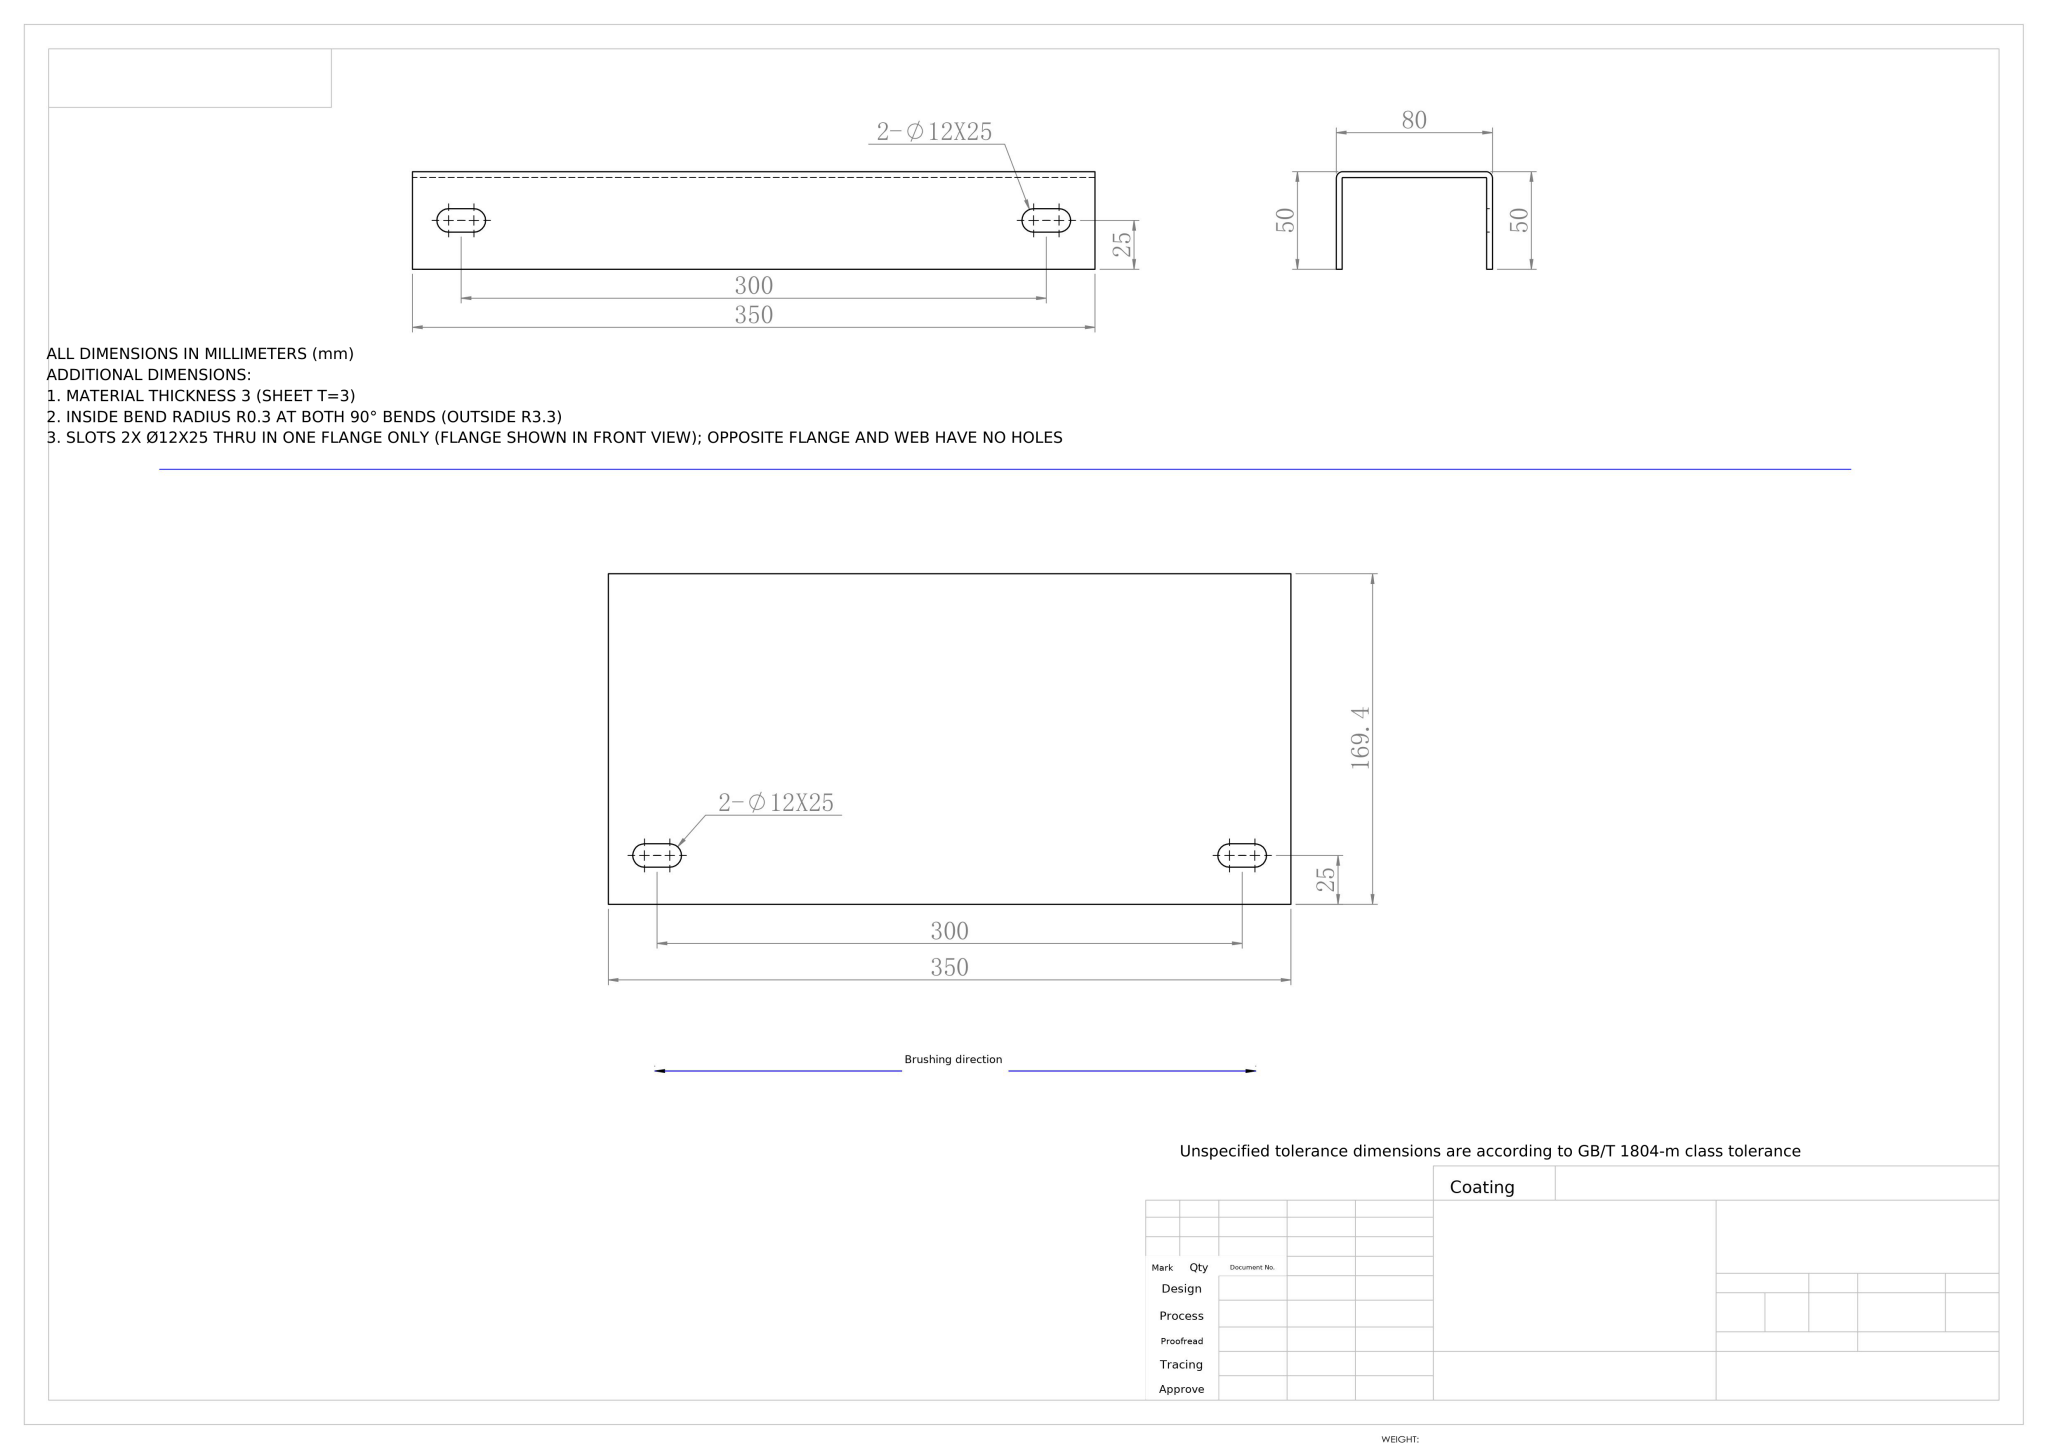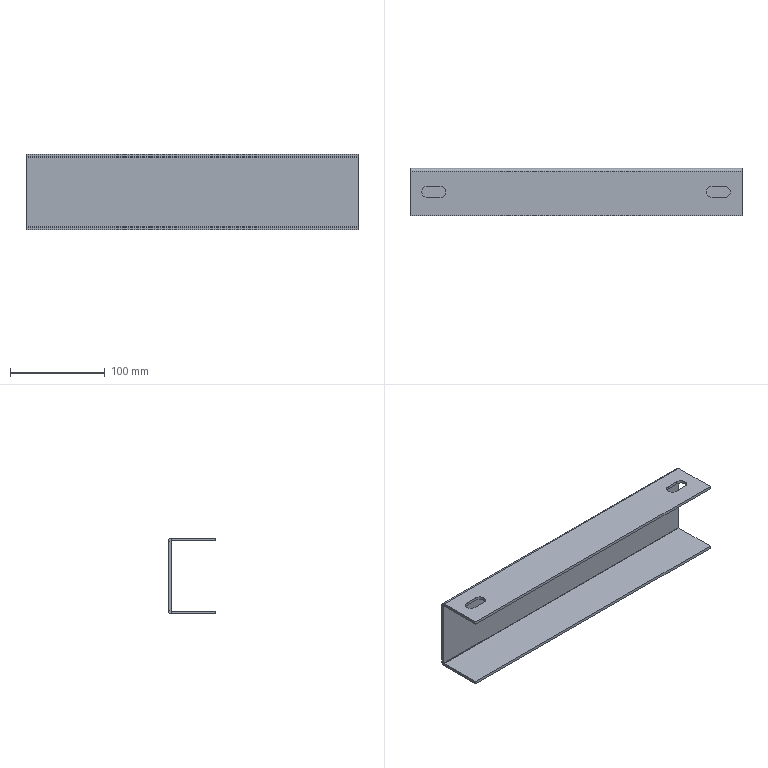Part | NX | mm | 1 solid | 32 faces | box 350 x 50 x 80 mm | volume 179463 mm3 | plane 22 | cylinder 10 | commonest cylinder face diameters 12 x6 6.6 x2 0.6 x2
STEP:
#1=COLOUR_RGB('',0.7529,0.7529,0.7529);
#2=FILL_AREA_STYLE_COLOUR('',#1);
#3=FILL_AREA_STYLE('',(#2));
#4=SURFACE_STYLE_FILL_AREA(#3);
#5=SURFACE_SIDE_STYLE('',(#4));
#6=SURFACE_STYLE_USAGE(.BOTH.,#5);
#7=PRESENTATION_STYLE_ASSIGNMENT((#6));
#8=CARTESIAN_POINT('',(337.5,25.,-3.));
#9=VERTEX_POINT('',#8);
#10=CARTESIAN_POINT('',(331.5,31.,-3.));
#11=VERTEX_POINT('',#10);
#12=CARTESIAN_POINT('',(331.5,25.,-3.));
#13=DIRECTION('',(0.,0.,1.));
#14=DIRECTION('',(-1.,0.,0.));
#15=AXIS2_PLACEMENT_3D('',#12,#13,#14);
#16=CIRCLE('',#15,6.);
#17=EDGE_CURVE('',#9,#11,#16,.T.);
#18=ORIENTED_EDGE('',*,*,#17,.F.);
#19=CARTESIAN_POINT('',(337.5,25.,0.));
#20=VERTEX_POINT('',#19);
#21=CARTESIAN_POINT('',(337.5,25.,-3.));
#22=DIRECTION('',(0.,0.,1.));
#23=VECTOR('',#22,1000.);
#24=LINE('',#21,#23);
#25=EDGE_CURVE('',#9,#20,#24,.T.);
#26=ORIENTED_EDGE('',*,*,#25,.T.);
#27=CARTESIAN_POINT('',(331.5,31.,0.));
#28=VERTEX_POINT('',#27);
#29=CARTESIAN_POINT('',(331.5,25.,0.));
#30=DIRECTION('',(0.,0.,1.));
#31=DIRECTION('',(-1.,0.,0.));
#32=AXIS2_PLACEMENT_3D('',#29,#30,#31);
#33=CIRCLE('',#32,6.);
#34=EDGE_CURVE('',#20,#28,#33,.T.);
#35=ORIENTED_EDGE('',*,*,#34,.T.);
#36=CARTESIAN_POINT('',(331.5,31.,-3.));
#37=DIRECTION('',(0.,0.,1.));
#38=VECTOR('',#37,1000.);
#39=LINE('',#36,#38);
#40=EDGE_CURVE('',#11,#28,#39,.T.);
#41=ORIENTED_EDGE('',*,*,#40,.F.);
#42=EDGE_LOOP('',(#18,#26,#35,#41));
#43=FACE_OUTER_BOUND('',#42,.T.);
#44=CARTESIAN_POINT('',(331.5,25.,-3.));
#45=DIRECTION('',(0.,0.,1.));
#46=DIRECTION('',(1.,0.,0.));
#47=AXIS2_PLACEMENT_3D('',#44,#45,#46);
#48=CYLINDRICAL_SURFACE('',#47,6.);
#49=ADVANCED_FACE('',(#43),#48,.F.);
#50=CARTESIAN_POINT('',(37.5,25.,-3.));
#51=VERTEX_POINT('',#50);
#52=CARTESIAN_POINT('',(31.5,31.,-3.));
#53=VERTEX_POINT('',#52);
#54=CARTESIAN_POINT('',(31.5,25.,-3.));
#55=DIRECTION('',(0.,0.,1.));
#56=DIRECTION('',(-1.,0.,0.));
#57=AXIS2_PLACEMENT_3D('',#54,#55,#56);
#58=CIRCLE('',#57,6.);
#59=EDGE_CURVE('',#51,#53,#58,.T.);
#60=ORIENTED_EDGE('',*,*,#59,.F.);
#61=CARTESIAN_POINT('',(37.5,25.,0.));
#62=VERTEX_POINT('',#61);
#63=CARTESIAN_POINT('',(37.5,25.,-3.));
#64=DIRECTION('',(0.,0.,1.));
#65=VECTOR('',#64,1000.);
#66=LINE('',#63,#65);
#67=EDGE_CURVE('',#51,#62,#66,.T.);
#68=ORIENTED_EDGE('',*,*,#67,.T.);
#69=CARTESIAN_POINT('',(31.5,31.,0.));
#70=VERTEX_POINT('',#69);
#71=CARTESIAN_POINT('',(31.5,25.,0.));
#72=DIRECTION('',(0.,0.,1.));
#73=DIRECTION('',(-1.,0.,0.));
#74=AXIS2_PLACEMENT_3D('',#71,#72,#73);
#75=CIRCLE('',#74,6.);
#76=EDGE_CURVE('',#62,#70,#75,.T.);
#77=ORIENTED_EDGE('',*,*,#76,.T.);
#78=CARTESIAN_POINT('',(31.5,31.,-3.));
#79=DIRECTION('',(0.,0.,1.));
#80=VECTOR('',#79,1000.);
#81=LINE('',#78,#80);
#82=EDGE_CURVE('',#53,#70,#81,.T.);
#83=ORIENTED_EDGE('',*,*,#82,.F.);
#84=EDGE_LOOP('',(#60,#68,#77,#83));
#85=FACE_OUTER_BOUND('',#84,.T.);
#86=CARTESIAN_POINT('',(31.5,25.,-3.));
#87=DIRECTION('',(0.,0.,1.));
#88=DIRECTION('',(1.,0.,0.));
#89=AXIS2_PLACEMENT_3D('',#86,#87,#88);
#90=CYLINDRICAL_SURFACE('',#89,6.);
#91=ADVANCED_FACE('',(#85),#90,.F.);
#92=CARTESIAN_POINT('',(350.,50.,-3.3));
#93=VERTEX_POINT('',#92);
#94=CARTESIAN_POINT('',(350.,47.,-3.3));
#95=VERTEX_POINT('',#94);
#96=CARTESIAN_POINT('',(350.,50.,-3.3));
#97=DIRECTION('',(0.,-1.,0.));
#98=VECTOR('',#97,1000.);
#99=LINE('',#96,#98);
#100=EDGE_CURVE('',#93,#95,#99,.T.);
#101=ORIENTED_EDGE('',*,*,#100,.F.);
#102=CARTESIAN_POINT('',(350.,46.7,0.));
#103=VERTEX_POINT('',#102);
#104=CARTESIAN_POINT('',(350.,46.7,-3.3));
#105=DIRECTION('',(-1.,0.,0.));
#106=DIRECTION('',(0.,0.,-1.));
#107=AXIS2_PLACEMENT_3D('',#104,#105,#106);
#108=CIRCLE('',#107,3.3);
#109=EDGE_CURVE('',#103,#93,#108,.T.);
#110=ORIENTED_EDGE('',*,*,#109,.F.);
#111=CARTESIAN_POINT('',(350.,46.7,-3.));
#112=VERTEX_POINT('',#111);
#113=CARTESIAN_POINT('',(350.,46.7,-3.));
#114=DIRECTION('',(0.,0.,1.));
#115=VECTOR('',#114,1000.);
#116=LINE('',#113,#115);
#117=EDGE_CURVE('',#112,#103,#116,.T.);
#118=ORIENTED_EDGE('',*,*,#117,.F.);
#119=CARTESIAN_POINT('',(350.,46.7,-3.3));
#120=DIRECTION('',(-1.,0.,0.));
#121=DIRECTION('',(0.,0.,-1.));
#122=AXIS2_PLACEMENT_3D('',#119,#120,#121);
#123=CIRCLE('',#122,0.3);
#124=EDGE_CURVE('',#112,#95,#123,.T.);
#125=ORIENTED_EDGE('',*,*,#124,.T.);
#126=EDGE_LOOP('',(#101,#110,#118,#125));
#127=FACE_OUTER_BOUND('',#126,.T.);
#128=CARTESIAN_POINT('',(350.,50.,-3.3));
#129=DIRECTION('',(1.,0.,0.));
#130=DIRECTION('',(0.,0.,-1.));
#131=AXIS2_PLACEMENT_3D('',#128,#129,#130);
#132=PLANE('',#131);
#133=ADVANCED_FACE('',(#127),#132,.T.);
#134=CARTESIAN_POINT('',(350.,50.,-76.7));
#135=VERTEX_POINT('',#134);
#136=CARTESIAN_POINT('',(350.,50.,0.));
#137=DIRECTION('',(0.,0.,-1.));
#138=VECTOR('',#137,1000.);
#139=LINE('',#136,#138);
#140=EDGE_CURVE('',#93,#135,#139,.T.);
#141=ORIENTED_EDGE('',*,*,#140,.F.);
#142=ORIENTED_EDGE('',*,*,#100,.T.);
#143=CARTESIAN_POINT('',(350.,47.,-76.7));
#144=VERTEX_POINT('',#143);
#145=CARTESIAN_POINT('',(350.,47.,0.));
#146=DIRECTION('',(0.,0.,-1.));
#147=VECTOR('',#146,1000.);
#148=LINE('',#145,#147);
#149=EDGE_CURVE('',#95,#144,#148,.T.);
#150=ORIENTED_EDGE('',*,*,#149,.T.);
#151=CARTESIAN_POINT('',(350.,47.,-76.7));
#152=DIRECTION('',(0.,1.,0.));
#153=VECTOR('',#152,1000.);
#154=LINE('',#151,#153);
#155=EDGE_CURVE('',#144,#135,#154,.T.);
#156=ORIENTED_EDGE('',*,*,#155,.T.);
#157=EDGE_LOOP('',(#141,#142,#150,#156));
#158=FACE_OUTER_BOUND('',#157,.T.);
#159=CARTESIAN_POINT('',(350.,46.7,-3.));
#160=DIRECTION('',(1.,0.,0.));
#161=DIRECTION('',(0.,0.,-1.));
#162=AXIS2_PLACEMENT_3D('',#159,#160,#161);
#163=PLANE('',#162);
#164=ADVANCED_FACE('',(#158),#163,.T.);
#165=CARTESIAN_POINT('',(0.,46.7,0.));
#166=VERTEX_POINT('',#165);
#167=CARTESIAN_POINT('',(0.,46.7,-3.));
#168=VERTEX_POINT('',#167);
#169=CARTESIAN_POINT('',(0.,46.7,0.));
#170=DIRECTION('',(0.,0.,-1.));
#171=VECTOR('',#170,1000.);
#172=LINE('',#169,#171);
#173=EDGE_CURVE('',#166,#168,#172,.T.);
#174=ORIENTED_EDGE('',*,*,#173,.F.);
#175=CARTESIAN_POINT('',(0.,50.,-3.3));
#176=VERTEX_POINT('',#175);
#177=CARTESIAN_POINT('',(0.,46.7,-3.3));
#178=DIRECTION('',(-1.,0.,0.));
#179=DIRECTION('',(0.,0.,-1.));
#180=AXIS2_PLACEMENT_3D('',#177,#178,#179);
#181=CIRCLE('',#180,3.3);
#182=EDGE_CURVE('',#166,#176,#181,.T.);
#183=ORIENTED_EDGE('',*,*,#182,.T.);
#184=CARTESIAN_POINT('',(0.,47.,-3.3));
#185=VERTEX_POINT('',#184);
#186=CARTESIAN_POINT('',(0.,47.,-3.3));
#187=DIRECTION('',(0.,1.,0.));
#188=VECTOR('',#187,1000.);
#189=LINE('',#186,#188);
#190=EDGE_CURVE('',#185,#176,#189,.T.);
#191=ORIENTED_EDGE('',*,*,#190,.F.);
#192=CARTESIAN_POINT('',(0.,46.7,-3.3));
#193=DIRECTION('',(-1.,0.,0.));
#194=DIRECTION('',(0.,0.,-1.));
#195=AXIS2_PLACEMENT_3D('',#192,#193,#194);
#196=CIRCLE('',#195,0.3);
#197=EDGE_CURVE('',#168,#185,#196,.T.);
#198=ORIENTED_EDGE('',*,*,#197,.F.);
#199=EDGE_LOOP('',(#174,#183,#191,#198));
#200=FACE_OUTER_BOUND('',#199,.T.);
#201=CARTESIAN_POINT('',(0.,46.7,0.));
#202=DIRECTION('',(-1.,0.,0.));
#203=DIRECTION('',(0.,0.,1.));
#204=AXIS2_PLACEMENT_3D('',#201,#202,#203);
#205=PLANE('',#204);
#206=ADVANCED_FACE('',(#200),#205,.T.);
#207=CARTESIAN_POINT('',(0.,0.,0.));
#208=VERTEX_POINT('',#207);
#209=CARTESIAN_POINT('',(0.,0.,0.));
#210=DIRECTION('',(0.,1.,0.));
#211=VECTOR('',#210,1000.);
#212=LINE('',#209,#211);
#213=EDGE_CURVE('',#208,#166,#212,.T.);
#214=ORIENTED_EDGE('',*,*,#213,.T.);
#215=ORIENTED_EDGE('',*,*,#173,.T.);
#216=CARTESIAN_POINT('',(0.,0.,-3.));
#217=VERTEX_POINT('',#216);
#218=CARTESIAN_POINT('',(0.,0.,-3.));
#219=DIRECTION('',(0.,1.,0.));
#220=VECTOR('',#219,1000.);
#221=LINE('',#218,#220);
#222=EDGE_CURVE('',#217,#168,#221,.T.);
#223=ORIENTED_EDGE('',*,*,#222,.F.);
#224=CARTESIAN_POINT('',(0.,0.,-3.));
#225=DIRECTION('',(0.,0.,1.));
#226=VECTOR('',#225,1000.);
#227=LINE('',#224,#226);
#228=EDGE_CURVE('',#217,#208,#227,.T.);
#229=ORIENTED_EDGE('',*,*,#228,.T.);
#230=EDGE_LOOP('',(#214,#215,#223,#229));
#231=FACE_OUTER_BOUND('',#230,.T.);
#232=CARTESIAN_POINT('',(0.,47.,-3.3));
#233=DIRECTION('',(-1.,0.,0.));
#234=DIRECTION('',(0.,0.,1.));
#235=AXIS2_PLACEMENT_3D('',#232,#233,#234);
#236=PLANE('',#235);
#237=ADVANCED_FACE('',(#231),#236,.T.);
#238=CARTESIAN_POINT('',(350.,46.7,-80.));
#239=VERTEX_POINT('',#238);
#240=CARTESIAN_POINT('',(350.,46.7,-77.));
#241=VERTEX_POINT('',#240);
#242=CARTESIAN_POINT('',(350.,46.7,-80.));
#243=DIRECTION('',(0.,0.,1.));
#244=VECTOR('',#243,1000.);
#245=LINE('',#242,#244);
#246=EDGE_CURVE('',#239,#241,#245,.T.);
#247=ORIENTED_EDGE('',*,*,#246,.F.);
#248=CARTESIAN_POINT('',(350.,46.7,-76.7));
#249=DIRECTION('',(-1.,0.,0.));
#250=DIRECTION('',(0.,0.,-1.));
#251=AXIS2_PLACEMENT_3D('',#248,#249,#250);
#252=CIRCLE('',#251,3.3);
#253=EDGE_CURVE('',#135,#239,#252,.T.);
#254=ORIENTED_EDGE('',*,*,#253,.F.);
#255=ORIENTED_EDGE('',*,*,#155,.F.);
#256=CARTESIAN_POINT('',(350.,46.7,-76.7));
#257=DIRECTION('',(-1.,0.,0.));
#258=DIRECTION('',(0.,0.,-1.));
#259=AXIS2_PLACEMENT_3D('',#256,#257,#258);
#260=CIRCLE('',#259,0.3);
#261=EDGE_CURVE('',#144,#241,#260,.T.);
#262=ORIENTED_EDGE('',*,*,#261,.T.);
#263=EDGE_LOOP('',(#247,#254,#255,#262));
#264=FACE_OUTER_BOUND('',#263,.T.);
#265=CARTESIAN_POINT('',(350.,46.7,-80.));
#266=DIRECTION('',(1.,0.,0.));
#267=DIRECTION('',(0.,0.,-1.));
#268=AXIS2_PLACEMENT_3D('',#265,#266,#267);
#269=PLANE('',#268);
#270=ADVANCED_FACE('',(#264),#269,.T.);
#271=CARTESIAN_POINT('',(350.,0.,-80.));
#272=VERTEX_POINT('',#271);
#273=CARTESIAN_POINT('',(350.,50.,-80.));
#274=DIRECTION('',(0.,-1.,0.));
#275=VECTOR('',#274,1000.);
#276=LINE('',#273,#275);
#277=EDGE_CURVE('',#239,#272,#276,.T.);
#278=ORIENTED_EDGE('',*,*,#277,.F.);
#279=ORIENTED_EDGE('',*,*,#246,.T.);
#280=CARTESIAN_POINT('',(350.,0.,-77.));
#281=VERTEX_POINT('',#280);
#282=CARTESIAN_POINT('',(350.,50.,-77.));
#283=DIRECTION('',(0.,-1.,0.));
#284=VECTOR('',#283,1000.);
#285=LINE('',#282,#284);
#286=EDGE_CURVE('',#241,#281,#285,.T.);
#287=ORIENTED_EDGE('',*,*,#286,.T.);
#288=CARTESIAN_POINT('',(350.,0.,-80.));
#289=DIRECTION('',(0.,0.,1.));
#290=VECTOR('',#289,1000.);
#291=LINE('',#288,#290);
#292=EDGE_CURVE('',#272,#281,#291,.T.);
#293=ORIENTED_EDGE('',*,*,#292,.F.);
#294=EDGE_LOOP('',(#278,#279,#287,#293));
#295=FACE_OUTER_BOUND('',#294,.T.);
#296=CARTESIAN_POINT('',(350.,47.,-76.7));
#297=DIRECTION('',(1.,0.,0.));
#298=DIRECTION('',(0.,0.,-1.));
#299=AXIS2_PLACEMENT_3D('',#296,#297,#298);
#300=PLANE('',#299);
#301=ADVANCED_FACE('',(#295),#300,.T.);
#302=CARTESIAN_POINT('',(0.,50.,-76.7));
#303=VERTEX_POINT('',#302);
#304=CARTESIAN_POINT('',(0.,47.,-76.7));
#305=VERTEX_POINT('',#304);
#306=CARTESIAN_POINT('',(0.,50.,-76.7));
#307=DIRECTION('',(0.,-1.,0.));
#308=VECTOR('',#307,1000.);
#309=LINE('',#306,#308);
#310=EDGE_CURVE('',#303,#305,#309,.T.);
#311=ORIENTED_EDGE('',*,*,#310,.F.);
#312=CARTESIAN_POINT('',(0.,46.7,-80.));
#313=VERTEX_POINT('',#312);
#314=CARTESIAN_POINT('',(0.,46.7,-76.7));
#315=DIRECTION('',(-1.,0.,0.));
#316=DIRECTION('',(0.,0.,-1.));
#317=AXIS2_PLACEMENT_3D('',#314,#315,#316);
#318=CIRCLE('',#317,3.3);
#319=EDGE_CURVE('',#303,#313,#318,.T.);
#320=ORIENTED_EDGE('',*,*,#319,.T.);
#321=CARTESIAN_POINT('',(0.,46.7,-77.));
#322=VERTEX_POINT('',#321);
#323=CARTESIAN_POINT('',(0.,46.7,-77.));
#324=DIRECTION('',(0.,0.,-1.));
#325=VECTOR('',#324,1000.);
#326=LINE('',#323,#325);
#327=EDGE_CURVE('',#322,#313,#326,.T.);
#328=ORIENTED_EDGE('',*,*,#327,.F.);
#329=CARTESIAN_POINT('',(0.,46.7,-76.7));
#330=DIRECTION('',(-1.,0.,0.));
#331=DIRECTION('',(0.,0.,-1.));
#332=AXIS2_PLACEMENT_3D('',#329,#330,#331);
#333=CIRCLE('',#332,0.3);
#334=EDGE_CURVE('',#305,#322,#333,.T.);
#335=ORIENTED_EDGE('',*,*,#334,.F.);
#336=EDGE_LOOP('',(#311,#320,#328,#335));
#337=FACE_OUTER_BOUND('',#336,.T.);
#338=CARTESIAN_POINT('',(0.,50.,-76.7));
#339=DIRECTION('',(-1.,0.,0.));
#340=DIRECTION('',(0.,0.,1.));
#341=AXIS2_PLACEMENT_3D('',#338,#339,#340);
#342=PLANE('',#341);
#343=ADVANCED_FACE('',(#337),#342,.T.);
#344=CARTESIAN_POINT('',(0.,50.,0.));
#345=DIRECTION('',(0.,0.,-1.));
#346=VECTOR('',#345,1000.);
#347=LINE('',#344,#346);
#348=EDGE_CURVE('',#176,#303,#347,.T.);
#349=ORIENTED_EDGE('',*,*,#348,.T.);
#350=ORIENTED_EDGE('',*,*,#310,.T.);
#351=CARTESIAN_POINT('',(0.,47.,0.));
#352=DIRECTION('',(0.,0.,-1.));
#353=VECTOR('',#352,1000.);
#354=LINE('',#351,#353);
#355=EDGE_CURVE('',#185,#305,#354,.T.);
#356=ORIENTED_EDGE('',*,*,#355,.F.);
#357=ORIENTED_EDGE('',*,*,#190,.T.);
#358=EDGE_LOOP('',(#349,#350,#356,#357));
#359=FACE_OUTER_BOUND('',#358,.T.);
#360=CARTESIAN_POINT('',(0.,46.7,-77.));
#361=DIRECTION('',(-1.,0.,0.));
#362=DIRECTION('',(0.,0.,1.));
#363=AXIS2_PLACEMENT_3D('',#360,#361,#362);
#364=PLANE('',#363);
#365=ADVANCED_FACE('',(#359),#364,.T.);
#366=CARTESIAN_POINT('',(0.,0.,-77.));
#367=VERTEX_POINT('',#366);
#368=CARTESIAN_POINT('',(0.,50.,-77.));
#369=DIRECTION('',(0.,-1.,0.));
#370=VECTOR('',#369,1000.);
#371=LINE('',#368,#370);
#372=EDGE_CURVE('',#322,#367,#371,.T.);
#373=ORIENTED_EDGE('',*,*,#372,.T.);
#374=CARTESIAN_POINT('',(350.,0.,-77.));
#375=DIRECTION('',(-1.,0.,0.));
#376=VECTOR('',#375,1000.);
#377=LINE('',#374,#376);
#378=EDGE_CURVE('',#281,#367,#377,.T.);
#379=ORIENTED_EDGE('',*,*,#378,.F.);
#380=ORIENTED_EDGE('',*,*,#286,.F.);
#381=CARTESIAN_POINT('',(350.,46.7,-77.));
#382=DIRECTION('',(-1.,0.,0.));
#383=VECTOR('',#382,1000.);
#384=LINE('',#381,#383);
#385=EDGE_CURVE('',#241,#322,#384,.T.);
#386=ORIENTED_EDGE('',*,*,#385,.T.);
#387=EDGE_LOOP('',(#373,#379,#380,#386));
#388=FACE_OUTER_BOUND('',#387,.T.);
#389=CARTESIAN_POINT('',(350.,50.,-77.));
#390=DIRECTION('',(0.,0.,-1.));
#391=DIRECTION('',(-1.,0.,0.));
#392=AXIS2_PLACEMENT_3D('',#389,#390,#391);
#393=PLANE('',#392);
#394=ADVANCED_FACE('',(#388),#393,.F.);
#395=CARTESIAN_POINT('',(0.,0.,-80.));
#396=VERTEX_POINT('',#395);
#397=CARTESIAN_POINT('',(0.,0.,-80.));
#398=DIRECTION('',(0.,0.,1.));
#399=VECTOR('',#398,1000.);
#400=LINE('',#397,#399);
#401=EDGE_CURVE('',#396,#367,#400,.T.);
#402=ORIENTED_EDGE('',*,*,#401,.F.);
#403=CARTESIAN_POINT('',(350.,0.,-80.));
#404=DIRECTION('',(-1.,0.,0.));
#405=VECTOR('',#404,1000.);
#406=LINE('',#403,#405);
#407=EDGE_CURVE('',#272,#396,#406,.T.);
#408=ORIENTED_EDGE('',*,*,#407,.F.);
#409=ORIENTED_EDGE('',*,*,#292,.T.);
#410=ORIENTED_EDGE('',*,*,#378,.T.);
#411=EDGE_LOOP('',(#402,#408,#409,#410));
#412=FACE_OUTER_BOUND('',#411,.T.);
#413=CARTESIAN_POINT('',(350.,0.,-80.));
#414=DIRECTION('',(0.,-1.,0.));
#415=DIRECTION('',(0.,0.,-1.));
#416=AXIS2_PLACEMENT_3D('',#413,#414,#415);
#417=PLANE('',#416);
#418=ADVANCED_FACE('',(#412),#417,.T.);
#419=CARTESIAN_POINT('',(0.,50.,-80.));
#420=DIRECTION('',(0.,-1.,0.));
#421=VECTOR('',#420,1000.);
#422=LINE('',#419,#421);
#423=EDGE_CURVE('',#313,#396,#422,.T.);
#424=ORIENTED_EDGE('',*,*,#423,.F.);
#425=CARTESIAN_POINT('',(350.,46.7,-80.));
#426=DIRECTION('',(-1.,0.,0.));
#427=VECTOR('',#426,1000.);
#428=LINE('',#425,#427);
#429=EDGE_CURVE('',#239,#313,#428,.T.);
#430=ORIENTED_EDGE('',*,*,#429,.F.);
#431=ORIENTED_EDGE('',*,*,#277,.T.);
#432=ORIENTED_EDGE('',*,*,#407,.T.);
#433=EDGE_LOOP('',(#424,#430,#431,#432));
#434=FACE_OUTER_BOUND('',#433,.T.);
#435=CARTESIAN_POINT('',(350.,50.,-80.));
#436=DIRECTION('',(0.,0.,-1.));
#437=DIRECTION('',(-1.,0.,0.));
#438=AXIS2_PLACEMENT_3D('',#435,#436,#437);
#439=PLANE('',#438);
#440=ADVANCED_FACE('',(#434),#439,.T.);
#441=ORIENTED_EDGE('',*,*,#319,.F.);
#442=CARTESIAN_POINT('',(350.,50.,-76.7));
#443=DIRECTION('',(-1.,0.,0.));
#444=VECTOR('',#443,1000.);
#445=LINE('',#442,#444);
#446=EDGE_CURVE('',#135,#303,#445,.T.);
#447=ORIENTED_EDGE('',*,*,#446,.F.);
#448=ORIENTED_EDGE('',*,*,#253,.T.);
#449=ORIENTED_EDGE('',*,*,#429,.T.);
#450=EDGE_LOOP('',(#441,#447,#448,#449));
#451=FACE_OUTER_BOUND('',#450,.T.);
#452=CARTESIAN_POINT('',(350.,46.7,-76.7));
#453=DIRECTION('',(-1.,0.,0.));
#454=DIRECTION('',(0.,0.,1.));
#455=AXIS2_PLACEMENT_3D('',#452,#453,#454);
#456=CYLINDRICAL_SURFACE('',#455,3.3);
#457=ADVANCED_FACE('',(#451),#456,.T.);
#458=ORIENTED_EDGE('',*,*,#348,.F.);
#459=CARTESIAN_POINT('',(350.,50.,-3.3));
#460=DIRECTION('',(-1.,0.,0.));
#461=VECTOR('',#460,1000.);
#462=LINE('',#459,#461);
#463=EDGE_CURVE('',#93,#176,#462,.T.);
#464=ORIENTED_EDGE('',*,*,#463,.F.);
#465=ORIENTED_EDGE('',*,*,#140,.T.);
#466=ORIENTED_EDGE('',*,*,#446,.T.);
#467=EDGE_LOOP('',(#458,#464,#465,#466));
#468=FACE_OUTER_BOUND('',#467,.T.);
#469=CARTESIAN_POINT('',(350.,50.,0.));
#470=DIRECTION('',(0.,1.,0.));
#471=DIRECTION('',(0.,0.,1.));
#472=AXIS2_PLACEMENT_3D('',#469,#470,#471);
#473=PLANE('',#472);
#474=ADVANCED_FACE('',(#468),#473,.T.);
#475=ORIENTED_EDGE('',*,*,#182,.F.);
#476=CARTESIAN_POINT('',(350.,46.7,0.));
#477=DIRECTION('',(-1.,0.,0.));
#478=VECTOR('',#477,1000.);
#479=LINE('',#476,#478);
#480=EDGE_CURVE('',#103,#166,#479,.T.);
#481=ORIENTED_EDGE('',*,*,#480,.F.);
#482=ORIENTED_EDGE('',*,*,#109,.T.);
#483=ORIENTED_EDGE('',*,*,#463,.T.);
#484=EDGE_LOOP('',(#475,#481,#482,#483));
#485=FACE_OUTER_BOUND('',#484,.T.);
#486=CARTESIAN_POINT('',(350.,46.7,-3.3));
#487=DIRECTION('',(-1.,0.,0.));
#488=DIRECTION('',(0.,0.,1.));
#489=AXIS2_PLACEMENT_3D('',#486,#487,#488);
#490=CYLINDRICAL_SURFACE('',#489,3.3);
#491=ADVANCED_FACE('',(#485),#490,.T.);
#492=CARTESIAN_POINT('',(331.5,19.,0.));
#493=VERTEX_POINT('',#492);
#494=CARTESIAN_POINT('',(331.5,25.,0.));
#495=DIRECTION('',(0.,0.,1.));
#496=DIRECTION('',(-1.,0.,0.));
#497=AXIS2_PLACEMENT_3D('',#494,#495,#496);
#498=CIRCLE('',#497,6.);
#499=EDGE_CURVE('',#493,#20,#498,.T.);
#500=ORIENTED_EDGE('',*,*,#499,.F.);
#501=CARTESIAN_POINT('',(318.5,19.,0.));
#502=VERTEX_POINT('',#501);
#503=CARTESIAN_POINT('',(331.5,19.,0.));
#504=DIRECTION('',(1.,0.,0.));
#505=VECTOR('',#504,1000.);
#506=LINE('',#503,#505);
#507=EDGE_CURVE('',#502,#493,#506,.T.);
#508=ORIENTED_EDGE('',*,*,#507,.F.);
#509=CARTESIAN_POINT('',(318.5,31.,0.));
#510=VERTEX_POINT('',#509);
#511=CARTESIAN_POINT('',(318.5,25.,0.));
#512=DIRECTION('',(0.,0.,1.));
#513=DIRECTION('',(1.,0.,0.));
#514=AXIS2_PLACEMENT_3D('',#511,#512,#513);
#515=CIRCLE('',#514,6.);
#516=EDGE_CURVE('',#510,#502,#515,.T.);
#517=ORIENTED_EDGE('',*,*,#516,.F.);
#518=CARTESIAN_POINT('',(331.5,31.,0.));
#519=DIRECTION('',(-1.,-0.,0.));
#520=VECTOR('',#519,1000.);
#521=LINE('',#518,#520);
#522=EDGE_CURVE('',#28,#510,#521,.T.);
#523=ORIENTED_EDGE('',*,*,#522,.F.);
#524=ORIENTED_EDGE('',*,*,#34,.F.);
#525=EDGE_LOOP('',(#500,#508,#517,#523,#524));
#526=FACE_BOUND('',#525,.T.);
#527=CARTESIAN_POINT('',(18.5,31.,0.));
#528=VERTEX_POINT('',#527);
#529=CARTESIAN_POINT('',(18.5,19.,0.));
#530=VERTEX_POINT('',#529);
#531=CARTESIAN_POINT('',(18.5,25.,0.));
#532=DIRECTION('',(0.,0.,1.));
#533=DIRECTION('',(1.,0.,0.));
#534=AXIS2_PLACEMENT_3D('',#531,#532,#533);
#535=CIRCLE('',#534,6.);
#536=EDGE_CURVE('',#528,#530,#535,.T.);
#537=ORIENTED_EDGE('',*,*,#536,.F.);
#538=CARTESIAN_POINT('',(18.5,31.,0.));
#539=DIRECTION('',(-1.,0.,0.));
#540=VECTOR('',#539,1000.);
#541=LINE('',#538,#540);
#542=EDGE_CURVE('',#70,#528,#541,.T.);
#543=ORIENTED_EDGE('',*,*,#542,.F.);
#544=ORIENTED_EDGE('',*,*,#76,.F.);
#545=CARTESIAN_POINT('',(31.5,19.,0.));
#546=VERTEX_POINT('',#545);
#547=CARTESIAN_POINT('',(31.5,25.,0.));
#548=DIRECTION('',(0.,0.,1.));
#549=DIRECTION('',(-1.,0.,0.));
#550=AXIS2_PLACEMENT_3D('',#547,#548,#549);
#551=CIRCLE('',#550,6.);
#552=EDGE_CURVE('',#546,#62,#551,.T.);
#553=ORIENTED_EDGE('',*,*,#552,.F.);
#554=CARTESIAN_POINT('',(18.5,19.,0.));
#555=DIRECTION('',(1.,0.,0.));
#556=VECTOR('',#555,1000.);
#557=LINE('',#554,#556);
#558=EDGE_CURVE('',#530,#546,#557,.T.);
#559=ORIENTED_EDGE('',*,*,#558,.F.);
#560=EDGE_LOOP('',(#537,#543,#544,#553,#559));
#561=FACE_BOUND('',#560,.T.);
#562=ORIENTED_EDGE('',*,*,#213,.F.);
#563=CARTESIAN_POINT('',(350.,0.,0.));
#564=VERTEX_POINT('',#563);
#565=CARTESIAN_POINT('',(350.,0.,0.));
#566=DIRECTION('',(-1.,0.,0.));
#567=VECTOR('',#566,1000.);
#568=LINE('',#565,#567);
#569=EDGE_CURVE('',#564,#208,#568,.T.);
#570=ORIENTED_EDGE('',*,*,#569,.F.);
#571=CARTESIAN_POINT('',(350.,0.,0.));
#572=DIRECTION('',(0.,1.,0.));
#573=VECTOR('',#572,1000.);
#574=LINE('',#571,#573);
#575=EDGE_CURVE('',#564,#103,#574,.T.);
#576=ORIENTED_EDGE('',*,*,#575,.T.);
#577=ORIENTED_EDGE('',*,*,#480,.T.);
#578=EDGE_LOOP('',(#562,#570,#576,#577));
#579=FACE_OUTER_BOUND('',#578,.T.);
#580=CARTESIAN_POINT('',(350.,0.,0.));
#581=DIRECTION('',(0.,0.,1.));
#582=DIRECTION('',(1.,0.,0.));
#583=AXIS2_PLACEMENT_3D('',#580,#581,#582);
#584=PLANE('',#583);
#585=ADVANCED_FACE('',(#526,#561,#579),#584,.T.);
#586=ORIENTED_EDGE('',*,*,#228,.F.);
#587=CARTESIAN_POINT('',(350.,0.,-3.));
#588=VERTEX_POINT('',#587);
#589=CARTESIAN_POINT('',(350.,0.,-3.));
#590=DIRECTION('',(-1.,0.,0.));
#591=VECTOR('',#590,1000.);
#592=LINE('',#589,#591);
#593=EDGE_CURVE('',#588,#217,#592,.T.);
#594=ORIENTED_EDGE('',*,*,#593,.F.);
#595=CARTESIAN_POINT('',(350.,0.,-3.));
#596=DIRECTION('',(0.,0.,1.));
#597=VECTOR('',#596,1000.);
#598=LINE('',#595,#597);
#599=EDGE_CURVE('',#588,#564,#598,.T.);
#600=ORIENTED_EDGE('',*,*,#599,.T.);
#601=ORIENTED_EDGE('',*,*,#569,.T.);
#602=EDGE_LOOP('',(#586,#594,#600,#601));
#603=FACE_OUTER_BOUND('',#602,.T.);
#604=CARTESIAN_POINT('',(350.,0.,-3.));
#605=DIRECTION('',(0.,-1.,0.));
#606=DIRECTION('',(0.,0.,-1.));
#607=AXIS2_PLACEMENT_3D('',#604,#605,#606);
#608=PLANE('',#607);
#609=ADVANCED_FACE('',(#603),#608,.T.);
#610=CARTESIAN_POINT('',(318.5,19.,-3.));
#611=VERTEX_POINT('',#610);
#612=CARTESIAN_POINT('',(331.5,19.,-3.));
#613=VERTEX_POINT('',#612);
#614=CARTESIAN_POINT('',(331.5,19.,-3.));
#615=DIRECTION('',(1.,0.,0.));
#616=VECTOR('',#615,1000.);
#617=LINE('',#614,#616);
#618=EDGE_CURVE('',#611,#613,#617,.T.);
#619=ORIENTED_EDGE('',*,*,#618,.T.);
#620=CARTESIAN_POINT('',(331.5,25.,-3.));
#621=DIRECTION('',(0.,0.,1.));
#622=DIRECTION('',(-1.,0.,0.));
#623=AXIS2_PLACEMENT_3D('',#620,#621,#622);
#624=CIRCLE('',#623,6.);
#625=EDGE_CURVE('',#613,#9,#624,.T.);
#626=ORIENTED_EDGE('',*,*,#625,.T.);
#627=ORIENTED_EDGE('',*,*,#17,.T.);
#628=CARTESIAN_POINT('',(318.5,31.,-3.));
#629=VERTEX_POINT('',#628);
#630=CARTESIAN_POINT('',(331.5,31.,-3.));
#631=DIRECTION('',(-1.,-0.,0.));
#632=VECTOR('',#631,1000.);
#633=LINE('',#630,#632);
#634=EDGE_CURVE('',#11,#629,#633,.T.);
#635=ORIENTED_EDGE('',*,*,#634,.T.);
#636=CARTESIAN_POINT('',(318.5,25.,-3.));
#637=DIRECTION('',(0.,0.,1.));
#638=DIRECTION('',(1.,0.,0.));
#639=AXIS2_PLACEMENT_3D('',#636,#637,#638);
#640=CIRCLE('',#639,6.);
#641=EDGE_CURVE('',#629,#611,#640,.T.);
#642=ORIENTED_EDGE('',*,*,#641,.T.);
#643=EDGE_LOOP('',(#619,#626,#627,#635,#642));
#644=FACE_BOUND('',#643,.T.);
#645=CARTESIAN_POINT('',(18.5,31.,-3.));
#646=VERTEX_POINT('',#645);
#647=CARTESIAN_POINT('',(18.5,31.,-3.));
#648=DIRECTION('',(-1.,0.,0.));
#649=VECTOR('',#648,1000.);
#650=LINE('',#647,#649);
#651=EDGE_CURVE('',#53,#646,#650,.T.);
#652=ORIENTED_EDGE('',*,*,#651,.T.);
#653=CARTESIAN_POINT('',(18.5,19.,-3.));
#654=VERTEX_POINT('',#653);
#655=CARTESIAN_POINT('',(18.5,25.,-3.));
#656=DIRECTION('',(0.,0.,1.));
#657=DIRECTION('',(1.,0.,0.));
#658=AXIS2_PLACEMENT_3D('',#655,#656,#657);
#659=CIRCLE('',#658,6.);
#660=EDGE_CURVE('',#646,#654,#659,.T.);
#661=ORIENTED_EDGE('',*,*,#660,.T.);
#662=CARTESIAN_POINT('',(31.5,19.,-3.));
#663=VERTEX_POINT('',#662);
#664=CARTESIAN_POINT('',(18.5,19.,-3.));
#665=DIRECTION('',(1.,0.,0.));
#666=VECTOR('',#665,1000.);
#667=LINE('',#664,#666);
#668=EDGE_CURVE('',#654,#663,#667,.T.);
#669=ORIENTED_EDGE('',*,*,#668,.T.);
#670=CARTESIAN_POINT('',(31.5,25.,-3.));
#671=DIRECTION('',(0.,0.,1.));
#672=DIRECTION('',(-1.,0.,0.));
#673=AXIS2_PLACEMENT_3D('',#670,#671,#672);
#674=CIRCLE('',#673,6.);
#675=EDGE_CURVE('',#663,#51,#674,.T.);
#676=ORIENTED_EDGE('',*,*,#675,.T.);
#677=ORIENTED_EDGE('',*,*,#59,.T.);
#678=EDGE_LOOP('',(#652,#661,#669,#676,#677));
#679=FACE_BOUND('',#678,.T.);
#680=ORIENTED_EDGE('',*,*,#222,.T.);
#681=CARTESIAN_POINT('',(350.,46.7,-3.));
#682=DIRECTION('',(-1.,0.,0.));
#683=VECTOR('',#682,1000.);
#684=LINE('',#681,#683);
#685=EDGE_CURVE('',#112,#168,#684,.T.);
#686=ORIENTED_EDGE('',*,*,#685,.F.);
#687=CARTESIAN_POINT('',(350.,0.,-3.));
#688=DIRECTION('',(0.,1.,0.));
#689=VECTOR('',#688,1000.);
#690=LINE('',#687,#689);
#691=EDGE_CURVE('',#588,#112,#690,.T.);
#692=ORIENTED_EDGE('',*,*,#691,.F.);
#693=ORIENTED_EDGE('',*,*,#593,.T.);
#694=EDGE_LOOP('',(#680,#686,#692,#693));
#695=FACE_OUTER_BOUND('',#694,.T.);
#696=CARTESIAN_POINT('',(350.,0.,-3.));
#697=DIRECTION('',(0.,0.,1.));
#698=DIRECTION('',(1.,0.,0.));
#699=AXIS2_PLACEMENT_3D('',#696,#697,#698);
#700=PLANE('',#699);
#701=ADVANCED_FACE('',(#644,#679,#695),#700,.F.);
#702=ORIENTED_EDGE('',*,*,#197,.T.);
#703=CARTESIAN_POINT('',(350.,47.,-3.3));
#704=DIRECTION('',(-1.,0.,0.));
#705=VECTOR('',#704,1000.);
#706=LINE('',#703,#705);
#707=EDGE_CURVE('',#95,#185,#706,.T.);
#708=ORIENTED_EDGE('',*,*,#707,.F.);
#709=ORIENTED_EDGE('',*,*,#124,.F.);
#710=ORIENTED_EDGE('',*,*,#685,.T.);
#711=EDGE_LOOP('',(#702,#708,#709,#710));
#712=FACE_OUTER_BOUND('',#711,.T.);
#713=CARTESIAN_POINT('',(350.,46.7,-3.3));
#714=DIRECTION('',(-1.,0.,0.));
#715=DIRECTION('',(0.,0.,1.));
#716=AXIS2_PLACEMENT_3D('',#713,#714,#715);
#717=CYLINDRICAL_SURFACE('',#716,0.3);
#718=ADVANCED_FACE('',(#712),#717,.F.);
#719=ORIENTED_EDGE('',*,*,#355,.T.);
#720=CARTESIAN_POINT('',(350.,47.,-76.7));
#721=DIRECTION('',(-1.,0.,0.));
#722=VECTOR('',#721,1000.);
#723=LINE('',#720,#722);
#724=EDGE_CURVE('',#144,#305,#723,.T.);
#725=ORIENTED_EDGE('',*,*,#724,.F.);
#726=ORIENTED_EDGE('',*,*,#149,.F.);
#727=ORIENTED_EDGE('',*,*,#707,.T.);
#728=EDGE_LOOP('',(#719,#725,#726,#727));
#729=FACE_OUTER_BOUND('',#728,.T.);
#730=CARTESIAN_POINT('',(350.,47.,0.));
#731=DIRECTION('',(0.,1.,0.));
#732=DIRECTION('',(0.,0.,1.));
#733=AXIS2_PLACEMENT_3D('',#730,#731,#732);
#734=PLANE('',#733);
#735=ADVANCED_FACE('',(#729),#734,.F.);
#736=ORIENTED_EDGE('',*,*,#334,.T.);
#737=ORIENTED_EDGE('',*,*,#385,.F.);
#738=ORIENTED_EDGE('',*,*,#261,.F.);
#739=ORIENTED_EDGE('',*,*,#724,.T.);
#740=EDGE_LOOP('',(#736,#737,#738,#739));
#741=FACE_OUTER_BOUND('',#740,.T.);
#742=CARTESIAN_POINT('',(350.,46.7,-76.7));
#743=DIRECTION('',(-1.,0.,0.));
#744=DIRECTION('',(0.,0.,1.));
#745=AXIS2_PLACEMENT_3D('',#742,#743,#744);
#746=CYLINDRICAL_SURFACE('',#745,0.3);
#747=ADVANCED_FACE('',(#741),#746,.F.);
#748=ORIENTED_EDGE('',*,*,#691,.T.);
#749=ORIENTED_EDGE('',*,*,#117,.T.);
#750=ORIENTED_EDGE('',*,*,#575,.F.);
#751=ORIENTED_EDGE('',*,*,#599,.F.);
#752=EDGE_LOOP('',(#748,#749,#750,#751));
#753=FACE_OUTER_BOUND('',#752,.T.);
#754=CARTESIAN_POINT('',(350.,46.7,-76.7));
#755=DIRECTION('',(1.,0.,0.));
#756=DIRECTION('',(0.,0.,-1.));
#757=AXIS2_PLACEMENT_3D('',#754,#755,#756);
#758=PLANE('',#757);
#759=ADVANCED_FACE('',(#753),#758,.T.);
#760=ORIENTED_EDGE('',*,*,#372,.F.);
#761=ORIENTED_EDGE('',*,*,#327,.T.);
#762=ORIENTED_EDGE('',*,*,#423,.T.);
#763=ORIENTED_EDGE('',*,*,#401,.T.);
#764=EDGE_LOOP('',(#760,#761,#762,#763));
#765=FACE_OUTER_BOUND('',#764,.T.);
#766=CARTESIAN_POINT('',(0.,46.7,-76.7));
#767=DIRECTION('',(1.,0.,0.));
#768=DIRECTION('',(0.,0.,-1.));
#769=AXIS2_PLACEMENT_3D('',#766,#767,#768);
#770=PLANE('',#769);
#771=ADVANCED_FACE('',(#765),#770,.F.);
#772=ORIENTED_EDGE('',*,*,#536,.T.);
#773=CARTESIAN_POINT('',(18.5,19.,-3.));
#774=DIRECTION('',(0.,0.,1.));
#775=VECTOR('',#774,1000.);
#776=LINE('',#773,#775);
#777=EDGE_CURVE('',#654,#530,#776,.T.);
#778=ORIENTED_EDGE('',*,*,#777,.F.);
#779=ORIENTED_EDGE('',*,*,#660,.F.);
#780=CARTESIAN_POINT('',(18.5,31.,-3.));
#781=DIRECTION('',(0.,0.,1.));
#782=VECTOR('',#781,1000.);
#783=LINE('',#780,#782);
#784=EDGE_CURVE('',#646,#528,#783,.T.);
#785=ORIENTED_EDGE('',*,*,#784,.T.);
#786=EDGE_LOOP('',(#772,#778,#779,#785));
#787=FACE_OUTER_BOUND('',#786,.T.);
#788=CARTESIAN_POINT('',(18.5,25.,-3.));
#789=DIRECTION('',(0.,0.,1.));
#790=DIRECTION('',(1.,0.,0.));
#791=AXIS2_PLACEMENT_3D('',#788,#789,#790);
#792=CYLINDRICAL_SURFACE('',#791,6.);
#793=ADVANCED_FACE('',(#787),#792,.F.);
#794=ORIENTED_EDGE('',*,*,#542,.T.);
#795=ORIENTED_EDGE('',*,*,#784,.F.);
#796=ORIENTED_EDGE('',*,*,#651,.F.);
#797=ORIENTED_EDGE('',*,*,#82,.T.);
#798=EDGE_LOOP('',(#794,#795,#796,#797));
#799=FACE_OUTER_BOUND('',#798,.T.);
#800=CARTESIAN_POINT('',(18.5,31.,-3.));
#801=DIRECTION('',(0.,1.,0.));
#802=DIRECTION('',(-1.,0.,0.));
#803=AXIS2_PLACEMENT_3D('',#800,#801,#802);
#804=PLANE('',#803);
#805=ADVANCED_FACE('',(#799),#804,.F.);
#806=ORIENTED_EDGE('',*,*,#67,.F.);
#807=ORIENTED_EDGE('',*,*,#675,.F.);
#808=CARTESIAN_POINT('',(31.5,19.,-3.));
#809=DIRECTION('',(0.,0.,1.));
#810=VECTOR('',#809,1000.);
#811=LINE('',#808,#810);
#812=EDGE_CURVE('',#663,#546,#811,.T.);
#813=ORIENTED_EDGE('',*,*,#812,.T.);
#814=ORIENTED_EDGE('',*,*,#552,.T.);
#815=EDGE_LOOP('',(#806,#807,#813,#814));
#816=FACE_OUTER_BOUND('',#815,.T.);
#817=CARTESIAN_POINT('',(31.5,25.,-3.));
#818=DIRECTION('',(0.,0.,1.));
#819=DIRECTION('',(1.,0.,0.));
#820=AXIS2_PLACEMENT_3D('',#817,#818,#819);
#821=CYLINDRICAL_SURFACE('',#820,6.);
#822=ADVANCED_FACE('',(#816),#821,.F.);
#823=ORIENTED_EDGE('',*,*,#558,.T.);
#824=ORIENTED_EDGE('',*,*,#812,.F.);
#825=ORIENTED_EDGE('',*,*,#668,.F.);
#826=ORIENTED_EDGE('',*,*,#777,.T.);
#827=EDGE_LOOP('',(#823,#824,#825,#826));
#828=FACE_OUTER_BOUND('',#827,.T.);
#829=CARTESIAN_POINT('',(18.5,19.,-3.));
#830=DIRECTION('',(0.,-1.,0.));
#831=DIRECTION('',(0.,0.,-1.));
#832=AXIS2_PLACEMENT_3D('',#829,#830,#831);
#833=PLANE('',#832);
#834=ADVANCED_FACE('',(#828),#833,.F.);
#835=ORIENTED_EDGE('',*,*,#25,.F.);
#836=ORIENTED_EDGE('',*,*,#625,.F.);
#837=CARTESIAN_POINT('',(331.5,19.,-3.));
#838=DIRECTION('',(0.,0.,1.));
#839=VECTOR('',#838,1000.);
#840=LINE('',#837,#839);
#841=EDGE_CURVE('',#613,#493,#840,.T.);
#842=ORIENTED_EDGE('',*,*,#841,.T.);
#843=ORIENTED_EDGE('',*,*,#499,.T.);
#844=EDGE_LOOP('',(#835,#836,#842,#843));
#845=FACE_OUTER_BOUND('',#844,.T.);
#846=CARTESIAN_POINT('',(331.5,25.,-3.));
#847=DIRECTION('',(0.,0.,1.));
#848=DIRECTION('',(1.,0.,0.));
#849=AXIS2_PLACEMENT_3D('',#846,#847,#848);
#850=CYLINDRICAL_SURFACE('',#849,6.);
#851=ADVANCED_FACE('',(#845),#850,.F.);
#852=ORIENTED_EDGE('',*,*,#507,.T.);
#853=ORIENTED_EDGE('',*,*,#841,.F.);
#854=ORIENTED_EDGE('',*,*,#618,.F.);
#855=CARTESIAN_POINT('',(318.5,19.,-3.));
#856=DIRECTION('',(0.,0.,1.));
#857=VECTOR('',#856,1000.);
#858=LINE('',#855,#857);
#859=EDGE_CURVE('',#611,#502,#858,.T.);
#860=ORIENTED_EDGE('',*,*,#859,.T.);
#861=EDGE_LOOP('',(#852,#853,#854,#860));
#862=FACE_OUTER_BOUND('',#861,.T.);
#863=CARTESIAN_POINT('',(331.5,19.,-3.));
#864=DIRECTION('',(0.,-1.,0.));
#865=DIRECTION('',(0.,0.,-1.));
#866=AXIS2_PLACEMENT_3D('',#863,#864,#865);
#867=PLANE('',#866);
#868=ADVANCED_FACE('',(#862),#867,.F.);
#869=ORIENTED_EDGE('',*,*,#516,.T.);
#870=ORIENTED_EDGE('',*,*,#859,.F.);
#871=ORIENTED_EDGE('',*,*,#641,.F.);
#872=CARTESIAN_POINT('',(318.5,31.,-3.));
#873=DIRECTION('',(0.,0.,1.));
#874=VECTOR('',#873,1000.);
#875=LINE('',#872,#874);
#876=EDGE_CURVE('',#629,#510,#875,.T.);
#877=ORIENTED_EDGE('',*,*,#876,.T.);
#878=EDGE_LOOP('',(#869,#870,#871,#877));
#879=FACE_OUTER_BOUND('',#878,.T.);
#880=CARTESIAN_POINT('',(318.5,25.,-3.));
#881=DIRECTION('',(0.,0.,1.));
#882=DIRECTION('',(1.,0.,0.));
#883=AXIS2_PLACEMENT_3D('',#880,#881,#882);
#884=CYLINDRICAL_SURFACE('',#883,6.);
#885=ADVANCED_FACE('',(#879),#884,.F.);
#886=ORIENTED_EDGE('',*,*,#522,.T.);
#887=ORIENTED_EDGE('',*,*,#876,.F.);
#888=ORIENTED_EDGE('',*,*,#634,.F.);
#889=ORIENTED_EDGE('',*,*,#40,.T.);
#890=EDGE_LOOP('',(#886,#887,#888,#889));
#891=FACE_OUTER_BOUND('',#890,.T.);
#892=CARTESIAN_POINT('',(331.5,31.,-3.));
#893=DIRECTION('',(-0.,1.,0.));
#894=DIRECTION('',(-1.,-0.,0.));
#895=AXIS2_PLACEMENT_3D('',#892,#893,#894);
#896=PLANE('',#895);
#897=ADVANCED_FACE('',(#891),#896,.F.);
#898=CLOSED_SHELL('',(#49,#91,#133,#164,#206,#237,#270,#301,#343,#365,#394,#418,#440,#457,#474,#491,#585,#609,#701,#718,#735,#747,#759,#771,#793,#805,#822,#834,#851,#868,#885,#897));
#899=MANIFOLD_SOLID_BREP('',#898);
#900=STYLED_ITEM('',(#7),#899);
#901=(LENGTH_UNIT()NAMED_UNIT(*)SI_UNIT(.MILLI.,.METRE.));
#902=UNCERTAINTY_MEASURE_WITH_UNIT(LENGTH_MEASURE(0.00001),#901,'','');
#903=(NAMED_UNIT(*)PLANE_ANGLE_UNIT()SI_UNIT($,.RADIAN.));
#904=(NAMED_UNIT(*)SI_UNIT($,.STERADIAN.)SOLID_ANGLE_UNIT());
#905=(GEOMETRIC_REPRESENTATION_CONTEXT(3)GLOBAL_UNCERTAINTY_ASSIGNED_CONTEXT((#902))GLOBAL_UNIT_ASSIGNED_CONTEXT((#901,#903,#904))REPRESENTATION_CONTEXT('',''));
#906=MECHANICAL_DESIGN_GEOMETRIC_PRESENTATION_REPRESENTATION('',(#900),#905);
#907=COLOUR_RGB('',0.7529,0.7529,0.7529);
#908=FILL_AREA_STYLE_COLOUR('',#907);
#909=FILL_AREA_STYLE('',(#908));
#910=SURFACE_STYLE_FILL_AREA(#909);
#911=SURFACE_SIDE_STYLE('',(#910));
#912=SURFACE_STYLE_USAGE(.BOTH.,#911);
#913=PRESENTATION_STYLE_ASSIGNMENT((#912));
#914=CARTESIAN_POINT('',(0.,0.,0.));
#915=DIRECTION('',(0.,0.,1.));
#916=DIRECTION('',(1.,0.,0.));
#917=AXIS2_PLACEMENT_3D('',#914,#915,#916);
#918=(LENGTH_UNIT()NAMED_UNIT(*)SI_UNIT(.MILLI.,.METRE.));
#919=UNCERTAINTY_MEASURE_WITH_UNIT(LENGTH_MEASURE(0.00001),#918,'','');
#920=(NAMED_UNIT(*)PLANE_ANGLE_UNIT()SI_UNIT($,.RADIAN.));
#921=(NAMED_UNIT(*)SI_UNIT($,.STERADIAN.)SOLID_ANGLE_UNIT());
#922=(GEOMETRIC_REPRESENTATION_CONTEXT(3)GLOBAL_UNCERTAINTY_ASSIGNED_CONTEXT((#919))GLOBAL_UNIT_ASSIGNED_CONTEXT((#918,#920,#921))REPRESENTATION_CONTEXT('',''));
#923=ADVANCED_BREP_SHAPE_REPRESENTATION('',(#899,#917),#922);
#924=STYLED_ITEM('',(#913),#923);
#925=(LENGTH_UNIT()NAMED_UNIT(*)SI_UNIT(.MILLI.,.METRE.));
#926=UNCERTAINTY_MEASURE_WITH_UNIT(LENGTH_MEASURE(0.00001),#925,'','');
#927=(NAMED_UNIT(*)PLANE_ANGLE_UNIT()SI_UNIT($,.RADIAN.));
#928=(NAMED_UNIT(*)SI_UNIT($,.STERADIAN.)SOLID_ANGLE_UNIT());
#929=(GEOMETRIC_REPRESENTATION_CONTEXT(3)GLOBAL_UNCERTAINTY_ASSIGNED_CONTEXT((#926))GLOBAL_UNIT_ASSIGNED_CONTEXT((#925,#927,#928))REPRESENTATION_CONTEXT('',''));
#930=MECHANICAL_DESIGN_GEOMETRIC_PRESENTATION_REPRESENTATION('',(#924),#929);
#931=PRESENTATION_LAYER_ASSIGNMENT('','',(#900));
#932=PRESENTATION_LAYER_ASSIGNMENT('','',(#924));